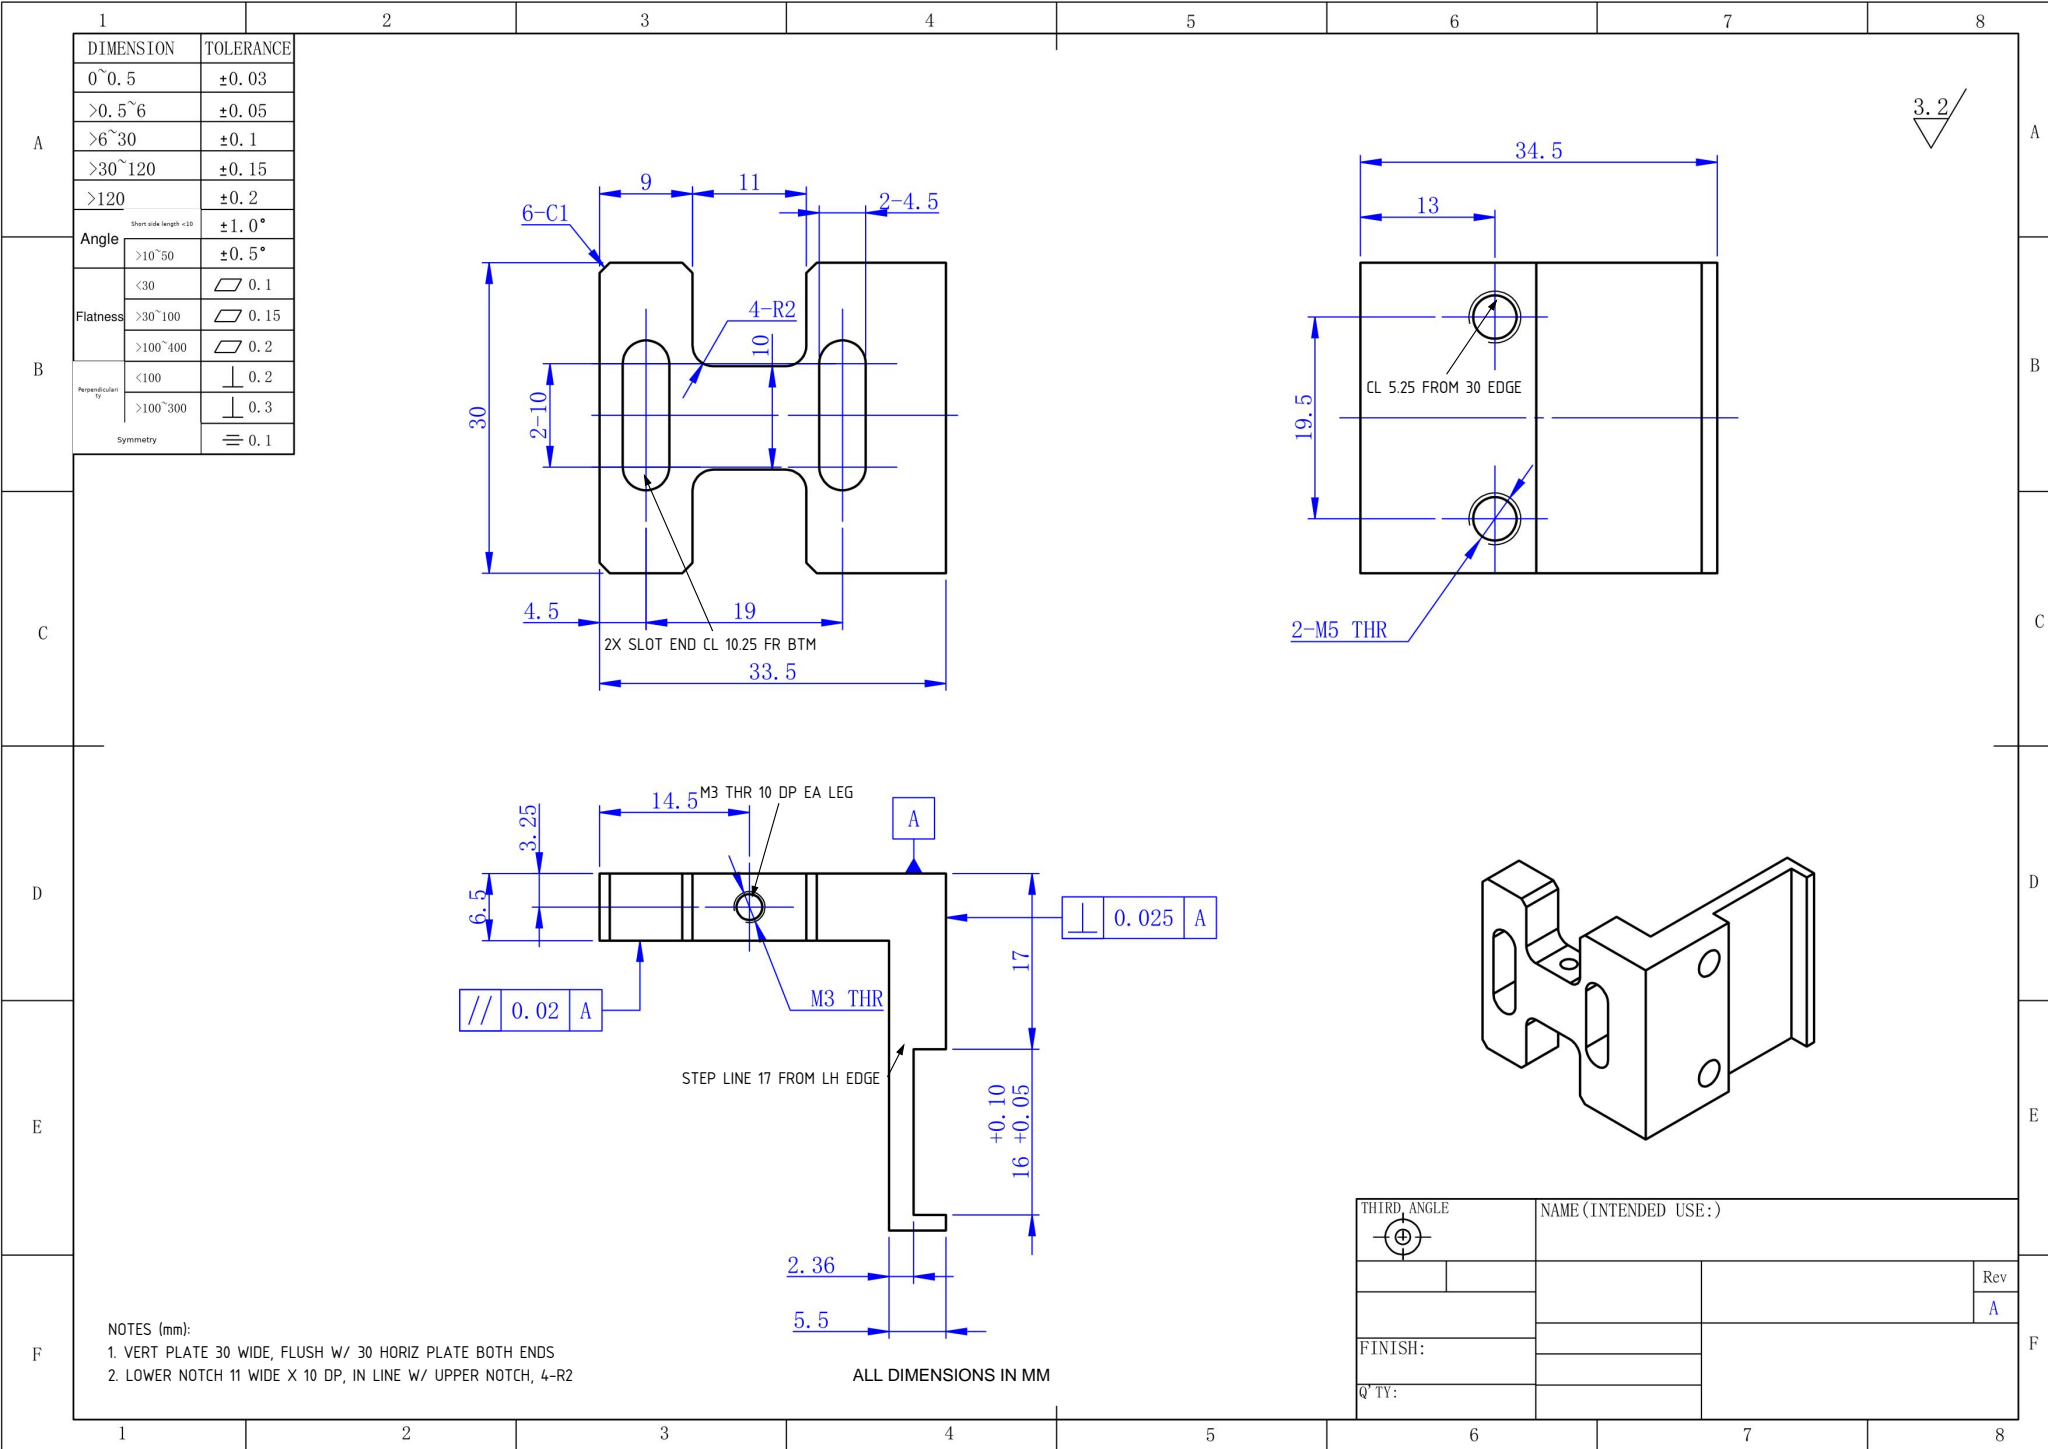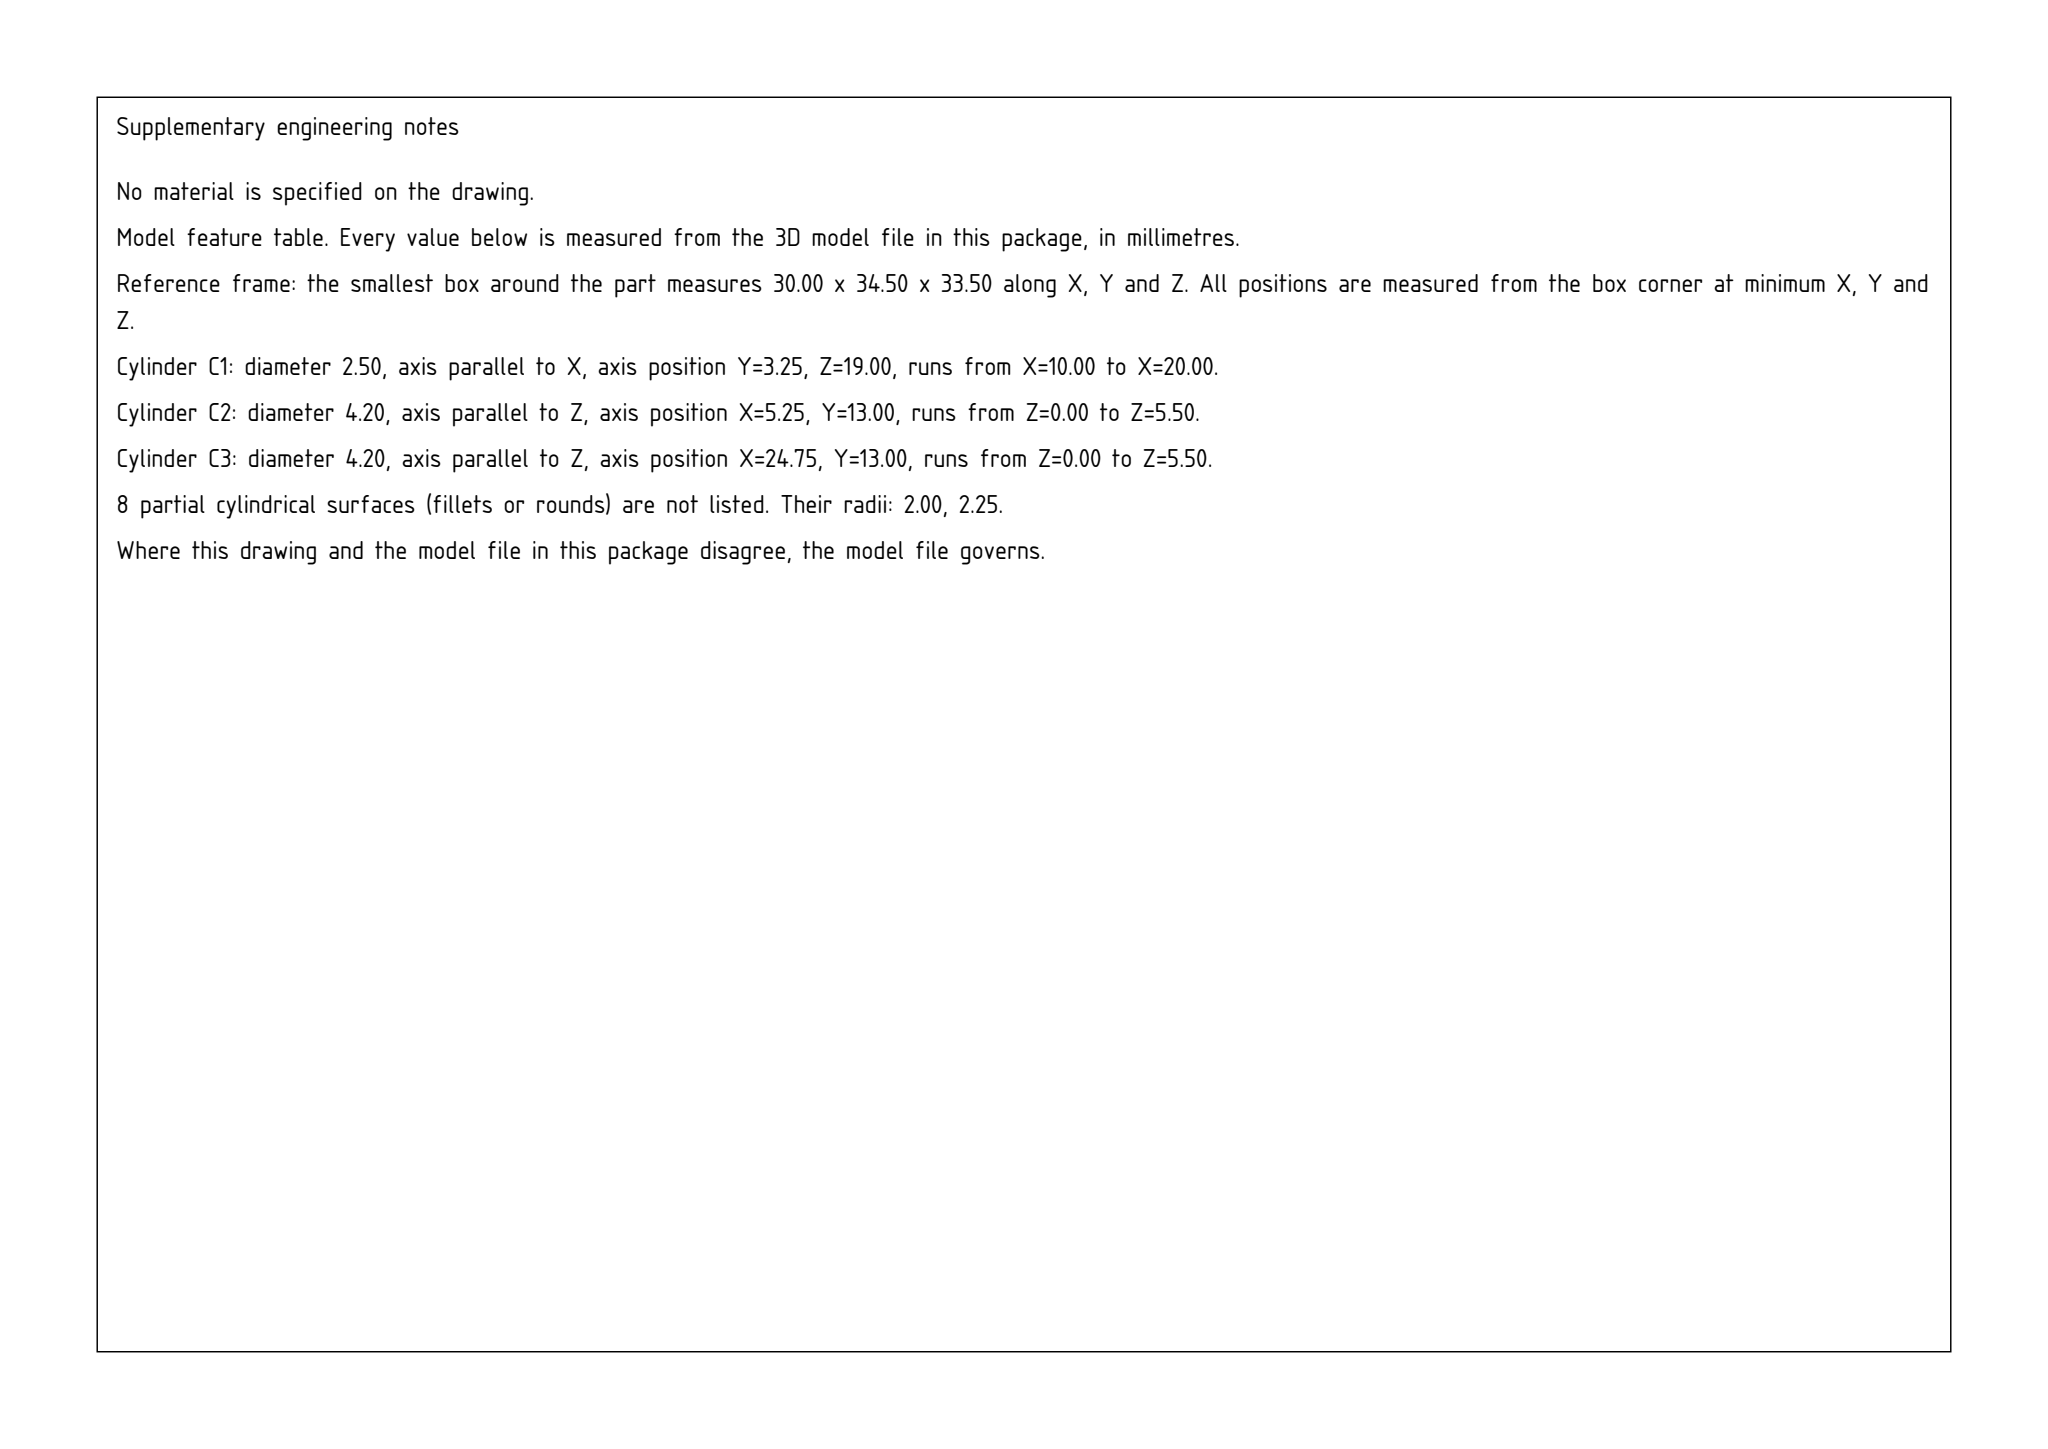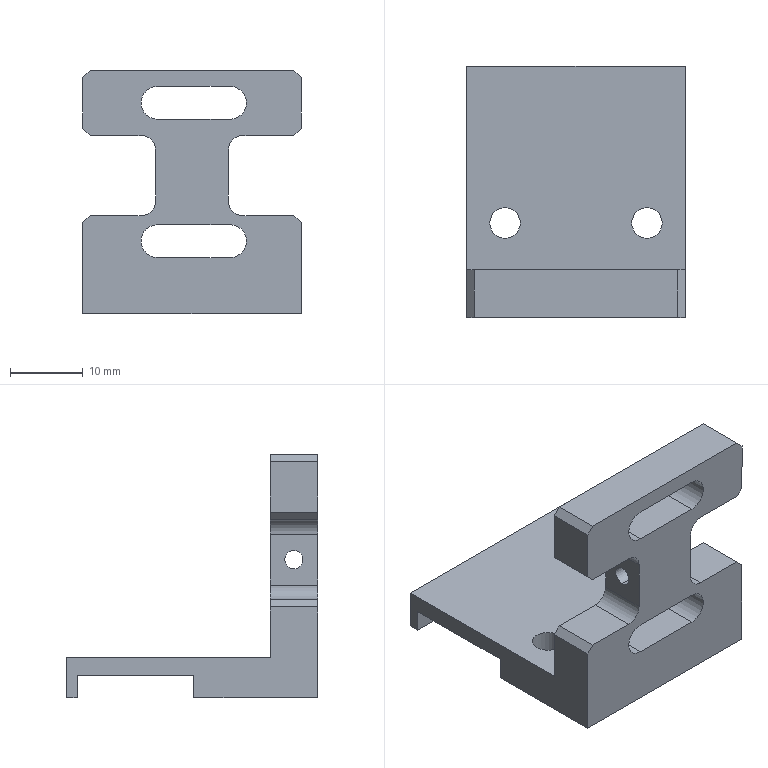Part | SolidWorks | mm | 1 solid | 44 faces | box 30 x 34.5 x 33.5 mm | volume 7225 mm3 | plane 30 | cylinder 14 | commonest cylinder face diameters 4.2 x4 4.5 x4 4 x4 2.5 x2
Drawing notes:
VERT PLATE 30 WIDE, FLUSH W/ 30 HORIZ PLATE BOTH ENDS | from the solid: X planes at 0.0 and 30.0 each count 2 (horiz + vert plate faces); bbox X = 30.0, no offset
STEP LINE 17 FROM LH EDGE: 5.5 THK TO 2.36 THK LIP | from the solid: Y planes 0, 17.0, 33.0, 34.5; Z 0/5.5 full thk, Z 3.14/5.5 lip 2.36 => step at y=17 from y=0
LOWER NOTCH 11 WIDE X 10 DP, IN LINE W/ UPPER NOTCH, 4-R2 | from the solid: Z planes 13.5 & 24.5 (count 2 ea) = 11 width; X planes 0/10 and 20/30 = 10 DP both notches
2-SLOT END R CL 10.25 FROM BTM & 9.75 FROM TOP OF 30 | from the solid: Ø4.5 Y-axis cyls at x=10.25 and x=20.25 (10 apart) in plate x 0..30
2-M5 THR IN 30 HIGH PLATE, CL 5.25 FROM EA 30 EDGE | from the solid: Ø4.2 Z-axis holes at x=5.25 and x=24.75 (19.5 apart), plate x 0..30, sym abt x=15
M3 THR THRU BOTH 10 WIDE LEGS, 10 DP EA, SYM ABT 30 CL | from the solid: Ø2.5 cyl, axis X, at y=3.25, z=19.0, length 10, count 2; X faces at 0,10,20,30